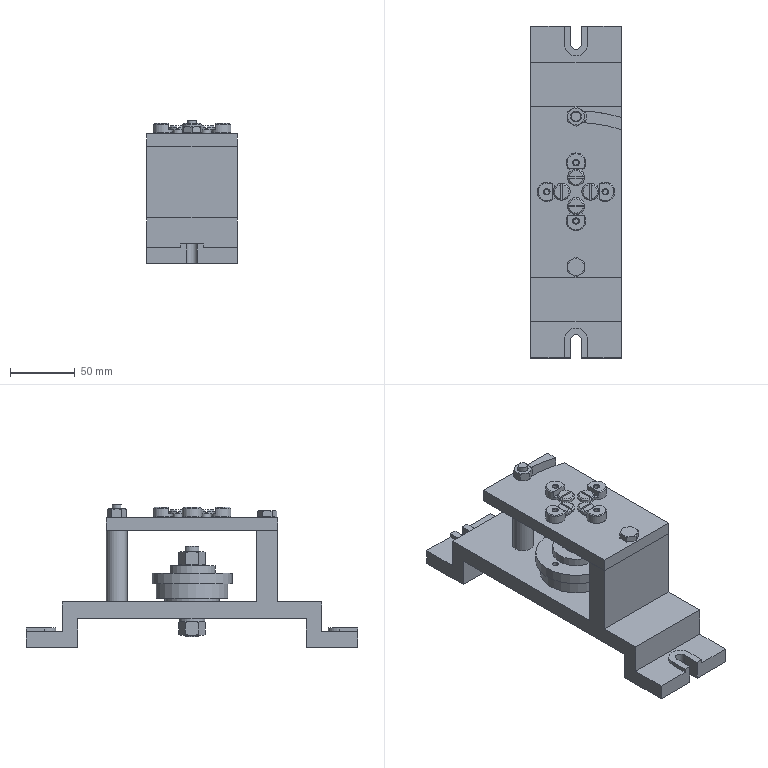Assembly | NX | mm | 20 component files | 20 solids | 335 faces | box 70 x 256 x 110 mm | volume 495756 mm3 | plane 166 | cone 88 | cylinder 78 | torus 3 | commonest cylinder face diameters 8 x11 4.2 x8 5 x8 13 x7 15 x4 4 x4 7.5 x4 18 x3
Bill of materials:
GB-T6170_F-2000,M8x1.25 | 1 |  | Hexagonal nut-like prism with a central through bore and chamfered/rounded corners on both end faces.
GB-T848-2002,M12 | 1 |  | Flat annular ring (plain washer-like disc): a thin circular plate with one concentric circular through-hole, flat parallel faces and a plain cylindrical outer edge.
unnamed part 1 | 4 |  | Revolved headed pin/screw-like part: wide disc head with a straight slot across its top, a cylindrical collar under the head, a narrower neck, and a cylindrical shank with a chamfered end.
GB-T5782-2000,M8x20 | 1 |  | Hexagon Head Bolt, GB-T 5782-2000,M8x20
unnamed part 2 | 1 |  | Flat circular disc of uniform thickness with a U-shaped slot running from the outer edge past the center (slotted/C-shaped washer form).
GB-T6171_T-2000,M12x1.5 | 1 |  | Hexagonal prism with a central circular through-bore (hex-nut-like body). Top corners are chamfered, the bore entry is chamfered or countersunk, and a short cylindrical step at the bottom is narrower than the hex.
unnamed part 3 | 1 |  | Solid stepped cylindrical pin: a long large-diameter main body, a shorter smaller-diameter step, a thin intermediate step or groove, and a small-diameter end spigot.
GB-T6170_F-2000,M12x1.75 | 1 |  | Hexagonal nut-like prism with a central through bore, countersunk bore entry, and chamfered corners on both end faces.
GB-T70.1-2000,M6x12 | 1 |  | Hexagon Socket Head Cap Screw, GB-T 70.1-2000,M6x12
unnamed part 4 | 1 |  | Flanged ring/bushing: thin circular flange with four equally spaced small through holes around a large central bore, plus a cylindrical spigot of slightly smaller diameter below the flange.
unnamed part 5 | 1 |  | Solid stepped shaft with a large central collar, a medium-diameter section on each side, and smaller end journals at both ends.
unnamed part 6 | 4 |  | Headed cylindrical pin with a small central through hole. One side of the head has a partial-depth flat cut, giving a D-shaped top. The head edges and the shank end are chamfered.
unnamed part 7 | 1 |  | Flat rectangular plate with a cross-shaped pattern of holes (four larger and four smaller), one additional hole near one end, and a curved slot open to the side edge near the opposite end.
unnamed part 8 | 1 |  | Elongated bracket with a hat-shaped (raised center) cross-section, a tall vertical wall/block rising from the raised top, open-ended slots in both end flanges, and several holes along the top.
Mates:
1. concentric | flange 1 edge | fixture_body 1 edge
2. concentric | mandrel 1 edge | flange 1 edge
3. concentric | C_washer 1 edge | flange 1 edge
4. concentric | GB-T6171_T-2000_M12x1_5 1 edge | C_washer 1 edge
5. concentric | GB-T848-2002_M12 1 edge | fixture_body 1 edge
6. concentric | GB-T6170_F-2000_M12x1_75 1 edge | GB-T848-2002_M12 1 edge
7. concentric | drill_template 1 edge | fixture_body 1 arc
8. concentric | drill_bushing 4 edge | drill_template 1 edge
9. concentric | drill_bushing_screw 4 edge | drill_template 1 edge
10. bond | mandrel 1 component | assembly component
11. bond | drill_bushing 4 component | assembly component
12. bond | drill_bushing_screw 4 component | assembly component
13. bond | drill_bushing 3 component | assembly component
14. bond | drill_bushing_screw 3 component | assembly component
15. bond | drill_bushing 2 component | assembly component
16. bond | drill_bushing_screw 2 component | assembly component
17. bond | drill_bushing 1 component | assembly component
18. bond | drill_bushing_screw 1 component | assembly component
19. circular | assembly datumaxis | assembly cartesiancoordinatesystem | assembly cartesiancoordinatesystem | assembly cartesiancoordinatesystem | assembly cartesiancoordinatesystem
20. circular | assembly datumaxis | assembly cartesiancoordinatesystem | assembly cartesiancoordinatesystem | assembly cartesiancoordinatesystem | assembly cartesiancoordinatesystem
21. concentric | support_rod 1 edge | drill_template 1 edge
22. concentric | GB-T6170_F-2000_M8x1_25 1 edge | drill_template 1 edge
23. fix | fixture_body 1 component